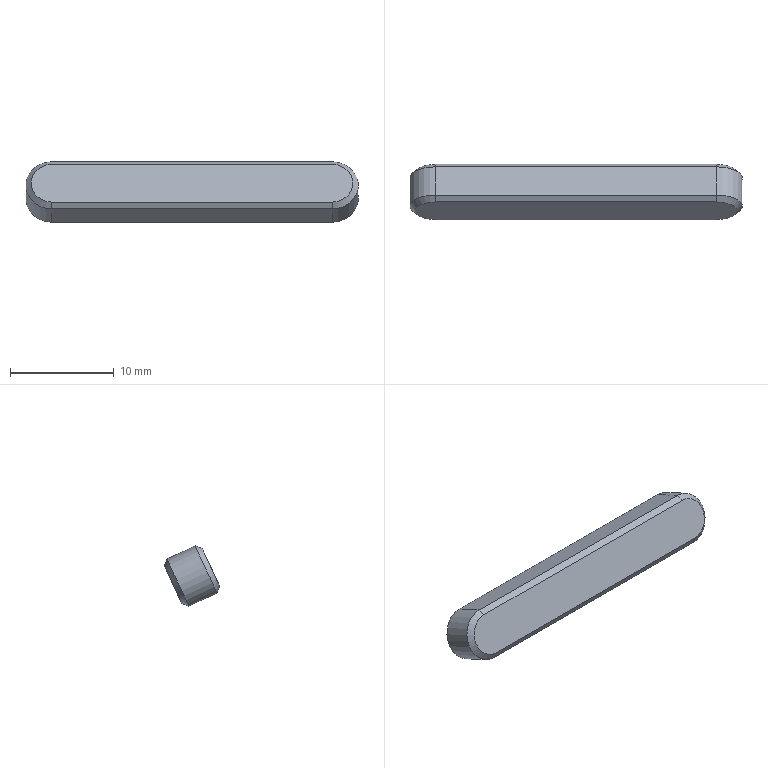Component | NX | KEY | 1 solid | 14 faces | box 32 x 5.32 x 5.8 mm | volume 601 mm3 | plane 8 | cone 4 | cylinder 2 | commonest cylinder face diameters 5 x2
STEP:
#1=CARTESIAN_POINT('',(0.,0.,0.));
#2=DIRECTION('',(0.,0.,1.));
#3=DIRECTION('',(1.,0.,0.));
#4=AXIS2_PLACEMENT_3D('',#1,#2,#3);
#5=CARTESIAN_POINT('',(56.5,-40.54,76.297));
#6=VERTEX_POINT('',#5);
#7=CARTESIAN_POINT('',(56.5,-43.259,77.565));
#8=VERTEX_POINT('',#7);
#9=CARTESIAN_POINT('',(56.5,-40.087,76.085));
#10=DIRECTION('',(0.,-0.9063,0.4226));
#11=VECTOR('',#10,1.);
#12=LINE('',#9,#11);
#13=CARTESIAN_POINT('',(56.5,-39.031,78.351));
#14=DIRECTION('',(0.,-0.9063,0.4226));
#15=DIRECTION('',(-1.,0.,0.));
#16=AXIS2_PLACEMENT_3D('',#13,#14,#15);
#17=CYLINDRICAL_SURFACE('',#16,2.5);
#18=CARTESIAN_POINT('',(1.571,-0.));
#19=DIRECTION('',(0.,1.));
#20=VECTOR('',#19,1.);
#21=LINE('',#18,#20);
#22=(GEOMETRIC_REPRESENTATION_CONTEXT(2)PARAMETRIC_REPRESENTATION_CONTEXT()REPRESENTATION_CONTEXT('',''));
#23=DEFINITIONAL_REPRESENTATION('',(#21),#22);
#24=PCURVE('',#17,#23);
#25=CARTESIAN_POINT('',(83.5,-40.087,76.085));
#26=DIRECTION('',(-0.,0.4226,0.9063));
#27=DIRECTION('',(1.,0.,0.));
#28=AXIS2_PLACEMENT_3D('',#25,#26,#27);
#29=PLANE('',#28);
#30=CARTESIAN_POINT('',(-27.,0.));
#31=DIRECTION('',(-0.,-1.));
#32=VECTOR('',#31,1.);
#33=LINE('',#30,#32);
#34=(GEOMETRIC_REPRESENTATION_CONTEXT(2)PARAMETRIC_REPRESENTATION_CONTEXT()REPRESENTATION_CONTEXT('',''));
#35=DEFINITIONAL_REPRESENTATION('',(#33),#34);
#36=PCURVE('',#29,#35);
#37=SURFACE_CURVE('',#12,(#24,#36),.PCURVE_S1.);
#38=EDGE_CURVE('',#6,#8,#37,.T.);
#39=ORIENTED_EDGE('',*,*,#38,.T.);
#40=CARTESIAN_POINT('',(56.5,-41.146,82.096));
#41=VERTEX_POINT('',#40);
#42=CARTESIAN_POINT('',(56.5,-42.203,79.83));
#43=DIRECTION('',(0.,0.9063,-0.4226));
#44=DIRECTION('',(1.,0.,0.));
#45=AXIS2_PLACEMENT_3D('',#42,#43,#44);
#46=CIRCLE('',#45,2.5);
#47=CARTESIAN_POINT('',(3.142,3.5));
#48=DIRECTION('',(-1.,0.));
#49=VECTOR('',#48,1.);
#50=LINE('',#47,#49);
#51=(GEOMETRIC_REPRESENTATION_CONTEXT(2)PARAMETRIC_REPRESENTATION_CONTEXT()REPRESENTATION_CONTEXT('',''));
#52=DEFINITIONAL_REPRESENTATION('',(#50),#51);
#53=PCURVE('',#17,#52);
#54=CARTESIAN_POINT('',(56.5,-42.203,79.83));
#55=DIRECTION('',(0.,0.9063,-0.4226));
#56=DIRECTION('',(1.,0.,0.));
#57=AXIS2_PLACEMENT_3D('',#54,#55,#56);
#58=CONICAL_SURFACE('',#57,2.5,0.7854);
#59=CARTESIAN_POINT('',(0.,0.));
#60=DIRECTION('',(1.,-0.));
#61=VECTOR('',#60,1.);
#62=LINE('',#59,#61);
#63=(GEOMETRIC_REPRESENTATION_CONTEXT(2)PARAMETRIC_REPRESENTATION_CONTEXT()REPRESENTATION_CONTEXT('',''));
#64=DEFINITIONAL_REPRESENTATION('',(#62),#63);
#65=PCURVE('',#58,#64);
#66=SURFACE_CURVE('',#46,(#53,#65),.PCURVE_S1.);
#67=EDGE_CURVE('',#8,#41,#66,.T.);
#68=ORIENTED_EDGE('',*,*,#67,.T.);
#69=CARTESIAN_POINT('',(56.5,-38.427,80.828));
#70=VERTEX_POINT('',#69);
#71=CARTESIAN_POINT('',(56.5,-37.974,80.617));
#72=DIRECTION('',(0.,-0.9063,0.4226));
#73=VECTOR('',#72,1.);
#74=LINE('',#71,#73);
#75=CARTESIAN_POINT('',(-1.571,-0.));
#76=DIRECTION('',(0.,1.));
#77=VECTOR('',#76,1.);
#78=LINE('',#75,#77);
#79=(GEOMETRIC_REPRESENTATION_CONTEXT(2)PARAMETRIC_REPRESENTATION_CONTEXT()REPRESENTATION_CONTEXT('',''));
#80=DEFINITIONAL_REPRESENTATION('',(#78),#79);
#81=PCURVE('',#17,#80);
#82=CARTESIAN_POINT('',(56.5,-37.974,80.617));
#83=DIRECTION('',(0.,-0.4226,-0.9063));
#84=DIRECTION('',(0.,0.9063,-0.4226));
#85=AXIS2_PLACEMENT_3D('',#82,#83,#84);
#86=PLANE('',#85);
#87=CARTESIAN_POINT('',(0.,0.));
#88=DIRECTION('',(-1.,0.));
#89=VECTOR('',#88,1.);
#90=LINE('',#87,#89);
#91=(GEOMETRIC_REPRESENTATION_CONTEXT(2)PARAMETRIC_REPRESENTATION_CONTEXT()REPRESENTATION_CONTEXT('',''));
#92=DEFINITIONAL_REPRESENTATION('',(#90),#91);
#93=PCURVE('',#86,#92);
#94=SURFACE_CURVE('',#74,(#81,#93),.PCURVE_S1.);
#95=EDGE_CURVE('',#70,#41,#94,.T.);
#96=ORIENTED_EDGE('',*,*,#95,.F.);
#97=CARTESIAN_POINT('',(56.5,-39.484,78.563));
#98=DIRECTION('',(0.,-0.9063,0.4226));
#99=DIRECTION('',(1.,0.,0.));
#100=AXIS2_PLACEMENT_3D('',#97,#98,#99);
#101=CIRCLE('',#100,2.5);
#102=CARTESIAN_POINT('',(-3.142,0.5));
#103=DIRECTION('',(1.,0.));
#104=VECTOR('',#103,1.);
#105=LINE('',#102,#104);
#106=(GEOMETRIC_REPRESENTATION_CONTEXT(2)PARAMETRIC_REPRESENTATION_CONTEXT()REPRESENTATION_CONTEXT('',''));
#107=DEFINITIONAL_REPRESENTATION('',(#105),#106);
#108=PCURVE('',#17,#107);
#109=CARTESIAN_POINT('',(56.5,-39.031,78.351));
#110=DIRECTION('',(0.,-0.9063,0.4226));
#111=DIRECTION('',(-1.,0.,0.));
#112=AXIS2_PLACEMENT_3D('',#109,#110,#111);
#113=CONICAL_SURFACE('',#112,2.,0.7854);
#114=CARTESIAN_POINT('',(-3.142,0.5));
#115=DIRECTION('',(1.,0.));
#116=VECTOR('',#115,1.);
#117=LINE('',#114,#116);
#118=(GEOMETRIC_REPRESENTATION_CONTEXT(2)PARAMETRIC_REPRESENTATION_CONTEXT()REPRESENTATION_CONTEXT('',''));
#119=DEFINITIONAL_REPRESENTATION('',(#117),#118);
#120=PCURVE('',#113,#119);
#121=SURFACE_CURVE('',#101,(#108,#120),.PCURVE_S1.);
#122=EDGE_CURVE('',#70,#6,#121,.T.);
#123=ORIENTED_EDGE('',*,*,#122,.T.);
#124=EDGE_LOOP('',(#39,#68,#96,#123));
#125=FACE_BOUND('',#124,.T.);
#126=ADVANCED_FACE('',(#125),#17,.T.);
#127=ORIENTED_EDGE('',*,*,#95,.T.);
#128=CARTESIAN_POINT('',(83.5,-41.146,82.096));
#129=VERTEX_POINT('',#128);
#130=CARTESIAN_POINT('',(56.5,-41.146,82.096));
#131=DIRECTION('',(1.,0.,0.));
#132=VECTOR('',#131,1.);
#133=LINE('',#130,#132);
#134=CARTESIAN_POINT('',(-3.5,0.));
#135=DIRECTION('',(0.,1.));
#136=VECTOR('',#135,1.);
#137=LINE('',#134,#136);
#138=(GEOMETRIC_REPRESENTATION_CONTEXT(2)PARAMETRIC_REPRESENTATION_CONTEXT()REPRESENTATION_CONTEXT('',''));
#139=DEFINITIONAL_REPRESENTATION('',(#137),#138);
#140=PCURVE('',#86,#139);
#141=CARTESIAN_POINT('',(56.5,-41.146,82.096));
#142=DIRECTION('',(0.,0.342,-0.9397));
#143=DIRECTION('',(1.,0.,0.));
#144=AXIS2_PLACEMENT_3D('',#141,#142,#143);
#145=PLANE('',#144);
#146=CARTESIAN_POINT('',(0.,0.));
#147=DIRECTION('',(1.,0.));
#148=VECTOR('',#147,1.);
#149=LINE('',#146,#148);
#150=(GEOMETRIC_REPRESENTATION_CONTEXT(2)PARAMETRIC_REPRESENTATION_CONTEXT()REPRESENTATION_CONTEXT('',''));
#151=DEFINITIONAL_REPRESENTATION('',(#149),#150);
#152=PCURVE('',#145,#151);
#153=SURFACE_CURVE('',#133,(#140,#152),.PCURVE_S1.);
#154=EDGE_CURVE('',#41,#129,#153,.T.);
#155=ORIENTED_EDGE('',*,*,#154,.T.);
#156=CARTESIAN_POINT('',(83.5,-38.427,80.828));
#157=VERTEX_POINT('',#156);
#158=CARTESIAN_POINT('',(83.5,-37.974,80.617));
#159=DIRECTION('',(0.,-0.9063,0.4226));
#160=VECTOR('',#159,1.);
#161=LINE('',#158,#160);
#162=CARTESIAN_POINT('',(0.,27.));
#163=DIRECTION('',(-1.,0.));
#164=VECTOR('',#163,1.);
#165=LINE('',#162,#164);
#166=(GEOMETRIC_REPRESENTATION_CONTEXT(2)PARAMETRIC_REPRESENTATION_CONTEXT()REPRESENTATION_CONTEXT('',''));
#167=DEFINITIONAL_REPRESENTATION('',(#165),#166);
#168=PCURVE('',#86,#167);
#169=CARTESIAN_POINT('',(83.5,-39.031,78.351));
#170=DIRECTION('',(0.,-0.9063,0.4226));
#171=DIRECTION('',(-1.,0.,0.));
#172=AXIS2_PLACEMENT_3D('',#169,#170,#171);
#173=CYLINDRICAL_SURFACE('',#172,2.5);
#174=CARTESIAN_POINT('',(4.712,-0.));
#175=DIRECTION('',(0.,1.));
#176=VECTOR('',#175,1.);
#177=LINE('',#174,#176);
#178=(GEOMETRIC_REPRESENTATION_CONTEXT(2)PARAMETRIC_REPRESENTATION_CONTEXT()REPRESENTATION_CONTEXT('',''));
#179=DEFINITIONAL_REPRESENTATION('',(#177),#178);
#180=PCURVE('',#173,#179);
#181=SURFACE_CURVE('',#161,(#168,#180),.PCURVE_S1.);
#182=EDGE_CURVE('',#157,#129,#181,.T.);
#183=ORIENTED_EDGE('',*,*,#182,.F.);
#184=CARTESIAN_POINT('',(56.5,-38.427,80.828));
#185=DIRECTION('',(-1.,0.,0.));
#186=VECTOR('',#185,1.);
#187=LINE('',#184,#186);
#188=CARTESIAN_POINT('',(-0.5,0.));
#189=DIRECTION('',(0.,-1.));
#190=VECTOR('',#189,1.);
#191=LINE('',#188,#190);
#192=(GEOMETRIC_REPRESENTATION_CONTEXT(2)PARAMETRIC_REPRESENTATION_CONTEXT()REPRESENTATION_CONTEXT('',''));
#193=DEFINITIONAL_REPRESENTATION('',(#191),#192);
#194=PCURVE('',#86,#193);
#195=CARTESIAN_POINT('',(56.5,-38.185,80.164));
#196=DIRECTION('',(0.,0.9397,0.342));
#197=DIRECTION('',(-1.,0.,0.));
#198=AXIS2_PLACEMENT_3D('',#195,#196,#197);
#199=PLANE('',#198);
#200=CARTESIAN_POINT('',(0.,0.7071));
#201=DIRECTION('',(1.,0.));
#202=VECTOR('',#201,1.);
#203=LINE('',#200,#202);
#204=(GEOMETRIC_REPRESENTATION_CONTEXT(2)PARAMETRIC_REPRESENTATION_CONTEXT()REPRESENTATION_CONTEXT('',''));
#205=DEFINITIONAL_REPRESENTATION('',(#203),#204);
#206=PCURVE('',#199,#205);
#207=SURFACE_CURVE('',#187,(#194,#206),.PCURVE_S1.);
#208=EDGE_CURVE('',#157,#70,#207,.T.);
#209=ORIENTED_EDGE('',*,*,#208,.T.);
#210=EDGE_LOOP('',(#127,#155,#183,#209));
#211=FACE_BOUND('',#210,.T.);
#212=ADVANCED_FACE('',(#211),#86,.F.);
#213=ORIENTED_EDGE('',*,*,#182,.T.);
#214=CARTESIAN_POINT('',(83.5,-43.259,77.565));
#215=VERTEX_POINT('',#214);
#216=CARTESIAN_POINT('',(83.5,-42.203,79.83));
#217=DIRECTION('',(0.,0.9063,-0.4226));
#218=DIRECTION('',(1.,0.,0.));
#219=AXIS2_PLACEMENT_3D('',#216,#217,#218);
#220=CIRCLE('',#219,2.5);
#221=CARTESIAN_POINT('',(9.425,3.5));
#222=DIRECTION('',(-1.,0.));
#223=VECTOR('',#222,1.);
#224=LINE('',#221,#223);
#225=(GEOMETRIC_REPRESENTATION_CONTEXT(2)PARAMETRIC_REPRESENTATION_CONTEXT()REPRESENTATION_CONTEXT('',''));
#226=DEFINITIONAL_REPRESENTATION('',(#224),#225);
#227=PCURVE('',#173,#226);
#228=CARTESIAN_POINT('',(83.5,-42.203,79.83));
#229=DIRECTION('',(0.,0.9063,-0.4226));
#230=DIRECTION('',(1.,0.,0.));
#231=AXIS2_PLACEMENT_3D('',#228,#229,#230);
#232=CONICAL_SURFACE('',#231,2.5,0.7854);
#233=CARTESIAN_POINT('',(0.,-0.));
#234=DIRECTION('',(1.,0.));
#235=VECTOR('',#234,1.);
#236=LINE('',#233,#235);
#237=(GEOMETRIC_REPRESENTATION_CONTEXT(2)PARAMETRIC_REPRESENTATION_CONTEXT()REPRESENTATION_CONTEXT('',''));
#238=DEFINITIONAL_REPRESENTATION('',(#236),#237);
#239=PCURVE('',#232,#238);
#240=SURFACE_CURVE('',#220,(#227,#239),.PCURVE_S1.);
#241=EDGE_CURVE('',#129,#215,#240,.T.);
#242=ORIENTED_EDGE('',*,*,#241,.T.);
#243=CARTESIAN_POINT('',(83.5,-40.54,76.297));
#244=VERTEX_POINT('',#243);
#245=CARTESIAN_POINT('',(83.5,-40.087,76.085));
#246=DIRECTION('',(0.,-0.9063,0.4226));
#247=VECTOR('',#246,1.);
#248=LINE('',#245,#247);
#249=CARTESIAN_POINT('',(1.571,-0.));
#250=DIRECTION('',(0.,1.));
#251=VECTOR('',#250,1.);
#252=LINE('',#249,#251);
#253=(GEOMETRIC_REPRESENTATION_CONTEXT(2)PARAMETRIC_REPRESENTATION_CONTEXT()REPRESENTATION_CONTEXT('',''));
#254=DEFINITIONAL_REPRESENTATION('',(#252),#253);
#255=PCURVE('',#173,#254);
#256=CARTESIAN_POINT('',(0.,0.));
#257=DIRECTION('',(-0.,-1.));
#258=VECTOR('',#257,1.);
#259=LINE('',#256,#258);
#260=(GEOMETRIC_REPRESENTATION_CONTEXT(2)PARAMETRIC_REPRESENTATION_CONTEXT()REPRESENTATION_CONTEXT('',''));
#261=DEFINITIONAL_REPRESENTATION('',(#259),#260);
#262=PCURVE('',#29,#261);
#263=SURFACE_CURVE('',#248,(#255,#262),.PCURVE_S1.);
#264=EDGE_CURVE('',#244,#215,#263,.T.);
#265=ORIENTED_EDGE('',*,*,#264,.F.);
#266=CARTESIAN_POINT('',(83.5,-39.484,78.563));
#267=DIRECTION('',(0.,-0.9063,0.4226));
#268=DIRECTION('',(1.,0.,0.));
#269=AXIS2_PLACEMENT_3D('',#266,#267,#268);
#270=CIRCLE('',#269,2.5);
#271=CARTESIAN_POINT('',(-3.142,0.5));
#272=DIRECTION('',(1.,0.));
#273=VECTOR('',#272,1.);
#274=LINE('',#271,#273);
#275=(GEOMETRIC_REPRESENTATION_CONTEXT(2)PARAMETRIC_REPRESENTATION_CONTEXT()REPRESENTATION_CONTEXT('',''));
#276=DEFINITIONAL_REPRESENTATION('',(#274),#275);
#277=PCURVE('',#173,#276);
#278=CARTESIAN_POINT('',(83.5,-39.031,78.351));
#279=DIRECTION('',(0.,-0.9063,0.4226));
#280=DIRECTION('',(-1.,0.,0.));
#281=AXIS2_PLACEMENT_3D('',#278,#279,#280);
#282=CONICAL_SURFACE('',#281,2.,0.7854);
#283=CARTESIAN_POINT('',(-3.142,0.5));
#284=DIRECTION('',(1.,-0.));
#285=VECTOR('',#284,1.);
#286=LINE('',#283,#285);
#287=(GEOMETRIC_REPRESENTATION_CONTEXT(2)PARAMETRIC_REPRESENTATION_CONTEXT()REPRESENTATION_CONTEXT('',''));
#288=DEFINITIONAL_REPRESENTATION('',(#286),#287);
#289=PCURVE('',#282,#288);
#290=SURFACE_CURVE('',#270,(#277,#289),.PCURVE_S1.);
#291=EDGE_CURVE('',#244,#157,#290,.T.);
#292=ORIENTED_EDGE('',*,*,#291,.T.);
#293=EDGE_LOOP('',(#213,#242,#265,#292));
#294=FACE_BOUND('',#293,.T.);
#295=ADVANCED_FACE('',(#294),#173,.T.);
#296=ORIENTED_EDGE('',*,*,#264,.T.);
#297=CARTESIAN_POINT('',(83.5,-43.259,77.565));
#298=DIRECTION('',(-1.,-0.,-0.));
#299=VECTOR('',#298,1.);
#300=LINE('',#297,#299);
#301=CARTESIAN_POINT('',(-0.,-3.5));
#302=DIRECTION('',(-1.,0.));
#303=VECTOR('',#302,1.);
#304=LINE('',#301,#303);
#305=(GEOMETRIC_REPRESENTATION_CONTEXT(2)PARAMETRIC_REPRESENTATION_CONTEXT()REPRESENTATION_CONTEXT('',''));
#306=DEFINITIONAL_REPRESENTATION('',(#304),#305);
#307=PCURVE('',#29,#306);
#308=CARTESIAN_POINT('',(83.5,-43.259,77.565));
#309=DIRECTION('',(-0.,0.9397,0.342));
#310=DIRECTION('',(-1.,-0.,-0.));
#311=AXIS2_PLACEMENT_3D('',#308,#309,#310);
#312=PLANE('',#311);
#313=CARTESIAN_POINT('',(0.,0.));
#314=DIRECTION('',(1.,-0.));
#315=VECTOR('',#314,1.);
#316=LINE('',#313,#315);
#317=(GEOMETRIC_REPRESENTATION_CONTEXT(2)PARAMETRIC_REPRESENTATION_CONTEXT()REPRESENTATION_CONTEXT('',''));
#318=DEFINITIONAL_REPRESENTATION('',(#316),#317);
#319=PCURVE('',#312,#318);
#320=SURFACE_CURVE('',#300,(#307,#319),.PCURVE_S1.);
#321=EDGE_CURVE('',#215,#8,#320,.T.);
#322=ORIENTED_EDGE('',*,*,#321,.T.);
#323=ORIENTED_EDGE('',*,*,#38,.F.);
#324=CARTESIAN_POINT('',(83.5,-40.54,76.297));
#325=DIRECTION('',(1.,0.,0.));
#326=VECTOR('',#325,1.);
#327=LINE('',#324,#326);
#328=CARTESIAN_POINT('',(-0.,-0.5));
#329=DIRECTION('',(1.,-0.));
#330=VECTOR('',#329,1.);
#331=LINE('',#328,#330);
#332=(GEOMETRIC_REPRESENTATION_CONTEXT(2)PARAMETRIC_REPRESENTATION_CONTEXT()REPRESENTATION_CONTEXT('',''));
#333=DEFINITIONAL_REPRESENTATION('',(#331),#332);
#334=PCURVE('',#29,#333);
#335=CARTESIAN_POINT('',(56.5,-39.876,76.539));
#336=DIRECTION('',(0.,0.342,-0.9397));
#337=DIRECTION('',(1.,0.,0.));
#338=AXIS2_PLACEMENT_3D('',#335,#336,#337);
#339=PLANE('',#338);
#340=CARTESIAN_POINT('',(27.,0.7071));
#341=DIRECTION('',(1.,-0.));
#342=VECTOR('',#341,1.);
#343=LINE('',#340,#342);
#344=(GEOMETRIC_REPRESENTATION_CONTEXT(2)PARAMETRIC_REPRESENTATION_CONTEXT()REPRESENTATION_CONTEXT('',''));
#345=DEFINITIONAL_REPRESENTATION('',(#343),#344);
#346=PCURVE('',#339,#345);
#347=SURFACE_CURVE('',#327,(#334,#346),.PCURVE_S1.);
#348=EDGE_CURVE('',#6,#244,#347,.T.);
#349=ORIENTED_EDGE('',*,*,#348,.T.);
#350=EDGE_LOOP('',(#296,#322,#323,#349));
#351=FACE_BOUND('',#350,.T.);
#352=ADVANCED_FACE('',(#351),#29,.F.);
#353=CARTESIAN_POINT('',(83.5,-39.876,76.539));
#354=VERTEX_POINT('',#353);
#355=CARTESIAN_POINT('',(56.5,-39.876,76.539));
#356=VERTEX_POINT('',#355);
#357=CARTESIAN_POINT('',(56.5,-39.876,76.539));
#358=DIRECTION('',(-1.,-0.,-0.));
#359=VECTOR('',#358,1.);
#360=LINE('',#357,#359);
#361=CARTESIAN_POINT('',(56.5,-39.031,78.351));
#362=DIRECTION('',(0.,0.9063,-0.4226));
#363=DIRECTION('',(1.,0.,0.));
#364=AXIS2_PLACEMENT_3D('',#361,#362,#363);
#365=PLANE('',#364);
#366=CARTESIAN_POINT('',(0.,2.));
#367=DIRECTION('',(-1.,0.));
#368=VECTOR('',#367,1.);
#369=LINE('',#366,#368);
#370=(GEOMETRIC_REPRESENTATION_CONTEXT(2)PARAMETRIC_REPRESENTATION_CONTEXT()REPRESENTATION_CONTEXT('',''));
#371=DEFINITIONAL_REPRESENTATION('',(#369),#370);
#372=PCURVE('',#365,#371);
#373=CARTESIAN_POINT('',(0.,0.));
#374=DIRECTION('',(-1.,0.));
#375=VECTOR('',#374,1.);
#376=LINE('',#373,#375);
#377=(GEOMETRIC_REPRESENTATION_CONTEXT(2)PARAMETRIC_REPRESENTATION_CONTEXT()REPRESENTATION_CONTEXT('',''));
#378=DEFINITIONAL_REPRESENTATION('',(#376),#377);
#379=PCURVE('',#339,#378);
#380=SURFACE_CURVE('',#360,(#372,#379),.PCURVE_S1.);
#381=EDGE_CURVE('',#354,#356,#380,.T.);
#382=ORIENTED_EDGE('',*,*,#381,.T.);
#383=CARTESIAN_POINT('',(56.5,-38.185,80.164));
#384=VERTEX_POINT('',#383);
#385=CARTESIAN_POINT('',(56.5,-39.031,78.351));
#386=DIRECTION('',(0.,0.9063,-0.4226));
#387=DIRECTION('',(1.,0.,0.));
#388=AXIS2_PLACEMENT_3D('',#385,#386,#387);
#389=CIRCLE('',#388,2.);
#390=CARTESIAN_POINT('',(0.,0.));
#391=DIRECTION('',(1.,0.));
#392=AXIS2_PLACEMENT_2D('',#390,#391);
#393=CIRCLE('',#392,2.);
#394=(GEOMETRIC_REPRESENTATION_CONTEXT(2)PARAMETRIC_REPRESENTATION_CONTEXT()REPRESENTATION_CONTEXT('',''));
#395=DEFINITIONAL_REPRESENTATION('',(#393),#394);
#396=PCURVE('',#365,#395);
#397=CARTESIAN_POINT('',(3.142,-0.));
#398=DIRECTION('',(-1.,0.));
#399=VECTOR('',#398,1.);
#400=LINE('',#397,#399);
#401=(GEOMETRIC_REPRESENTATION_CONTEXT(2)PARAMETRIC_REPRESENTATION_CONTEXT()REPRESENTATION_CONTEXT('',''));
#402=DEFINITIONAL_REPRESENTATION('',(#400),#401);
#403=PCURVE('',#113,#402);
#404=SURFACE_CURVE('',#389,(#396,#403),.PCURVE_S1.);
#405=EDGE_CURVE('',#356,#384,#404,.T.);
#406=ORIENTED_EDGE('',*,*,#405,.T.);
#407=CARTESIAN_POINT('',(83.5,-38.185,80.164));
#408=VERTEX_POINT('',#407);
#409=CARTESIAN_POINT('',(83.5,-38.185,80.164));
#410=DIRECTION('',(1.,0.,0.));
#411=VECTOR('',#410,1.);
#412=LINE('',#409,#411);
#413=CARTESIAN_POINT('',(27.,-2.));
#414=DIRECTION('',(1.,0.));
#415=VECTOR('',#414,1.);
#416=LINE('',#413,#415);
#417=(GEOMETRIC_REPRESENTATION_CONTEXT(2)PARAMETRIC_REPRESENTATION_CONTEXT()REPRESENTATION_CONTEXT('',''));
#418=DEFINITIONAL_REPRESENTATION('',(#416),#417);
#419=PCURVE('',#365,#418);
#420=CARTESIAN_POINT('',(-27.,0.));
#421=DIRECTION('',(-1.,0.));
#422=VECTOR('',#421,1.);
#423=LINE('',#420,#422);
#424=(GEOMETRIC_REPRESENTATION_CONTEXT(2)PARAMETRIC_REPRESENTATION_CONTEXT()REPRESENTATION_CONTEXT('',''));
#425=DEFINITIONAL_REPRESENTATION('',(#423),#424);
#426=PCURVE('',#199,#425);
#427=SURFACE_CURVE('',#412,(#419,#426),.PCURVE_S1.);
#428=EDGE_CURVE('',#384,#408,#427,.T.);
#429=ORIENTED_EDGE('',*,*,#428,.T.);
#430=CARTESIAN_POINT('',(83.5,-39.031,78.351));
#431=DIRECTION('',(0.,0.9063,-0.4226));
#432=DIRECTION('',(1.,0.,0.));
#433=AXIS2_PLACEMENT_3D('',#430,#431,#432);
#434=CIRCLE('',#433,2.);
#435=CARTESIAN_POINT('',(27.,0.));
#436=DIRECTION('',(1.,0.));
#437=AXIS2_PLACEMENT_2D('',#435,#436);
#438=CIRCLE('',#437,2.);
#439=(GEOMETRIC_REPRESENTATION_CONTEXT(2)PARAMETRIC_REPRESENTATION_CONTEXT()REPRESENTATION_CONTEXT('',''));
#440=DEFINITIONAL_REPRESENTATION('',(#438),#439);
#441=PCURVE('',#365,#440);
#442=CARTESIAN_POINT('',(9.425,-0.));
#443=DIRECTION('',(-1.,0.));
#444=VECTOR('',#443,1.);
#445=LINE('',#442,#444);
#446=(GEOMETRIC_REPRESENTATION_CONTEXT(2)PARAMETRIC_REPRESENTATION_CONTEXT()REPRESENTATION_CONTEXT('',''));
#447=DEFINITIONAL_REPRESENTATION('',(#445),#446);
#448=PCURVE('',#282,#447);
#449=SURFACE_CURVE('',#434,(#441,#448),.PCURVE_S1.);
#450=EDGE_CURVE('',#408,#354,#449,.T.);
#451=ORIENTED_EDGE('',*,*,#450,.T.);
#452=EDGE_LOOP('',(#382,#406,#429,#451));
#453=FACE_BOUND('',#452,.T.);
#454=ADVANCED_FACE('',(#453),#365,.T.);
#455=CARTESIAN_POINT('',(83.5,-41.811,81.854));
#456=VERTEX_POINT('',#455);
#457=CARTESIAN_POINT('',(56.5,-41.811,81.854));
#458=VERTEX_POINT('',#457);
#459=CARTESIAN_POINT('',(56.5,-41.811,81.854));
#460=DIRECTION('',(-1.,0.,0.));
#461=VECTOR('',#460,1.);
#462=LINE('',#459,#461);
#463=CARTESIAN_POINT('',(56.5,-42.656,80.042));
#464=DIRECTION('',(0.,0.9063,-0.4226));
#465=DIRECTION('',(1.,0.,0.));
#466=AXIS2_PLACEMENT_3D('',#463,#464,#465);
#467=PLANE('',#466);
#468=CARTESIAN_POINT('',(0.,-2.));
#469=DIRECTION('',(-1.,0.));
#470=VECTOR('',#469,1.);
#471=LINE('',#468,#470);
#472=(GEOMETRIC_REPRESENTATION_CONTEXT(2)PARAMETRIC_REPRESENTATION_CONTEXT()REPRESENTATION_CONTEXT('',''));
#473=DEFINITIONAL_REPRESENTATION('',(#471),#472);
#474=PCURVE('',#467,#473);
#475=CARTESIAN_POINT('',(0.,0.7071));
#476=DIRECTION('',(-1.,0.));
#477=VECTOR('',#476,1.);
#478=LINE('',#475,#477);
#479=(GEOMETRIC_REPRESENTATION_CONTEXT(2)PARAMETRIC_REPRESENTATION_CONTEXT()REPRESENTATION_CONTEXT('',''));
#480=DEFINITIONAL_REPRESENTATION('',(#478),#479);
#481=PCURVE('',#145,#480);
#482=SURFACE_CURVE('',#462,(#474,#481),.PCURVE_S1.);
#483=EDGE_CURVE('',#456,#458,#482,.T.);
#484=ORIENTED_EDGE('',*,*,#483,.T.);
#485=CARTESIAN_POINT('',(56.5,-43.501,78.229));
#486=VERTEX_POINT('',#485);
#487=CARTESIAN_POINT('',(56.5,-42.656,80.042));
#488=DIRECTION('',(0.,-0.9063,0.4226));
#489=DIRECTION('',(1.,0.,0.));
#490=AXIS2_PLACEMENT_3D('',#487,#488,#489);
#491=CIRCLE('',#490,2.);
#492=CARTESIAN_POINT('',(2.,0.));
#493=CARTESIAN_POINT('',(2.,-3.464));
#494=CARTESIAN_POINT('',(-1.,-1.732));
#495=CARTESIAN_POINT('',(-4.,-0.));
#496=CARTESIAN_POINT('',(-1.,1.732));
#497=CARTESIAN_POINT('',(2.,3.464));
#498=CARTESIAN_POINT('',(2.,0.));
#499=(BOUNDED_CURVE()B_SPLINE_CURVE(2,(#492,#493,#494,#495,#496,#497,#498),.UNSPECIFIED.,.T.,.F.)B_SPLINE_CURVE_WITH_KNOTS((1,2,2,2,2,1),(-2.094,0.,2.094,4.189,6.283,8.378),.UNSPECIFIED.)CURVE()GEOMETRIC_REPRESENTATION_ITEM()RATIONAL_B_SPLINE_CURVE((1.,0.5,1.,0.5,1.,0.5,1.))REPRESENTATION_ITEM(''));
#500=(GEOMETRIC_REPRESENTATION_CONTEXT(2)PARAMETRIC_REPRESENTATION_CONTEXT()REPRESENTATION_CONTEXT('',''));
#501=DEFINITIONAL_REPRESENTATION('',(#499),#500);
#502=PCURVE('',#467,#501);
#503=CARTESIAN_POINT('',(6.283,-0.5));
#504=DIRECTION('',(-1.,0.));
#505=VECTOR('',#504,1.);
#506=LINE('',#503,#505);
#507=(GEOMETRIC_REPRESENTATION_CONTEXT(2)PARAMETRIC_REPRESENTATION_CONTEXT()REPRESENTATION_CONTEXT('',''));
#508=DEFINITIONAL_REPRESENTATION('',(#506),#507);
#509=PCURVE('',#58,#508);
#510=SURFACE_CURVE('',#491,(#502,#509),.PCURVE_S1.);
#511=EDGE_CURVE('',#458,#486,#510,.T.);
#512=ORIENTED_EDGE('',*,*,#511,.T.);
#513=CARTESIAN_POINT('',(83.5,-43.501,78.229));
#514=VERTEX_POINT('',#513);
#515=CARTESIAN_POINT('',(56.5,-43.501,78.229));
#516=DIRECTION('',(1.,0.,0.));
#517=VECTOR('',#516,1.);
#518=LINE('',#515,#517);
#519=CARTESIAN_POINT('',(0.,2.));
#520=DIRECTION('',(1.,-0.));
#521=VECTOR('',#520,1.);
#522=LINE('',#519,#521);
#523=(GEOMETRIC_REPRESENTATION_CONTEXT(2)PARAMETRIC_REPRESENTATION_CONTEXT()REPRESENTATION_CONTEXT('',''));
#524=DEFINITIONAL_REPRESENTATION('',(#522),#523);
#525=PCURVE('',#467,#524);
#526=CARTESIAN_POINT('',(27.,0.7071));
#527=DIRECTION('',(-1.,0.));
#528=VECTOR('',#527,1.);
#529=LINE('',#526,#528);
#530=(GEOMETRIC_REPRESENTATION_CONTEXT(2)PARAMETRIC_REPRESENTATION_CONTEXT()REPRESENTATION_CONTEXT('',''));
#531=DEFINITIONAL_REPRESENTATION('',(#529),#530);
#532=PCURVE('',#312,#531);
#533=SURFACE_CURVE('',#518,(#525,#532),.PCURVE_S1.);
#534=EDGE_CURVE('',#486,#514,#533,.T.);
#535=ORIENTED_EDGE('',*,*,#534,.T.);
#536=CARTESIAN_POINT('',(83.5,-42.656,80.042));
#537=DIRECTION('',(0.,-0.9063,0.4226));
#538=DIRECTION('',(1.,0.,0.));
#539=AXIS2_PLACEMENT_3D('',#536,#537,#538);
#540=CIRCLE('',#539,2.);
#541=CARTESIAN_POINT('',(29.,0.));
#542=CARTESIAN_POINT('',(29.,-3.464));
#543=CARTESIAN_POINT('',(26.,-1.732));
#544=CARTESIAN_POINT('',(23.,-0.));
#545=CARTESIAN_POINT('',(26.,1.732));
#546=CARTESIAN_POINT('',(29.,3.464));
#547=CARTESIAN_POINT('',(29.,0.));
#548=(BOUNDED_CURVE()B_SPLINE_CURVE(2,(#541,#542,#543,#544,#545,#546,#547),.UNSPECIFIED.,.T.,.F.)B_SPLINE_CURVE_WITH_KNOTS((1,2,2,2,2,1),(-2.094,0.,2.094,4.189,6.283,8.378),.UNSPECIFIED.)CURVE()GEOMETRIC_REPRESENTATION_ITEM()RATIONAL_B_SPLINE_CURVE((1.,0.5,1.,0.5,1.,0.5,1.))REPRESENTATION_ITEM(''));
#549=(GEOMETRIC_REPRESENTATION_CONTEXT(2)PARAMETRIC_REPRESENTATION_CONTEXT()REPRESENTATION_CONTEXT('',''));
#550=DEFINITIONAL_REPRESENTATION('',(#548),#549);
#551=PCURVE('',#467,#550);
#552=CARTESIAN_POINT('',(12.566,-0.5));
#553=DIRECTION('',(-1.,-0.));
#554=VECTOR('',#553,1.);
#555=LINE('',#552,#554);
#556=(GEOMETRIC_REPRESENTATION_CONTEXT(2)PARAMETRIC_REPRESENTATION_CONTEXT()REPRESENTATION_CONTEXT('',''));
#557=DEFINITIONAL_REPRESENTATION('',(#555),#556);
#558=PCURVE('',#232,#557);
#559=SURFACE_CURVE('',#540,(#551,#558),.PCURVE_S1.);
#560=EDGE_CURVE('',#514,#456,#559,.T.);
#561=ORIENTED_EDGE('',*,*,#560,.T.);
#562=EDGE_LOOP('',(#484,#512,#535,#561));
#563=FACE_BOUND('',#562,.T.);
#564=ADVANCED_FACE('',(#563),#467,.F.);
#565=CARTESIAN_POINT('',(83.5,-41.811,81.854));
#566=DIRECTION('',(0.,0.9397,0.342));
#567=VECTOR('',#566,1.);
#568=LINE('',#565,#567);
#569=CARTESIAN_POINT('',(4.712,-0.5));
#570=DIRECTION('',(0.,1.));
#571=VECTOR('',#570,1.);
#572=LINE('',#569,#571);
#573=(GEOMETRIC_REPRESENTATION_CONTEXT(2)PARAMETRIC_REPRESENTATION_CONTEXT()REPRESENTATION_CONTEXT('',''));
#574=DEFINITIONAL_REPRESENTATION('',(#572),#573);
#575=PCURVE('',#232,#574);
#576=CARTESIAN_POINT('',(27.,0.7071));
#577=DIRECTION('',(0.,-1.));
#578=VECTOR('',#577,1.);
#579=LINE('',#576,#578);
#580=(GEOMETRIC_REPRESENTATION_CONTEXT(2)PARAMETRIC_REPRESENTATION_CONTEXT()REPRESENTATION_CONTEXT('',''));
#581=DEFINITIONAL_REPRESENTATION('',(#579),#580);
#582=PCURVE('',#145,#581);
#583=SURFACE_CURVE('',#568,(#575,#582),.PCURVE_S1.);
#584=EDGE_CURVE('',#456,#129,#583,.T.);
#585=ORIENTED_EDGE('',*,*,#584,.F.);
#586=ORIENTED_EDGE('',*,*,#560,.F.);
#587=CARTESIAN_POINT('',(83.5,-43.259,77.565));
#588=DIRECTION('',(0.,-0.342,0.9397));
#589=VECTOR('',#588,1.);
#590=LINE('',#587,#589);
#591=CARTESIAN_POINT('',(7.854,-0.));
#592=DIRECTION('',(0.,-1.));
#593=VECTOR('',#592,1.);
#594=LINE('',#591,#593);
#595=(GEOMETRIC_REPRESENTATION_CONTEXT(2)PARAMETRIC_REPRESENTATION_CONTEXT()REPRESENTATION_CONTEXT('',''));
#596=DEFINITIONAL_REPRESENTATION('',(#594),#595);
#597=PCURVE('',#232,#596);
#598=CARTESIAN_POINT('',(0.,0.));
#599=DIRECTION('',(-0.,1.));
#600=VECTOR('',#599,1.);
#601=LINE('',#598,#600);
#602=(GEOMETRIC_REPRESENTATION_CONTEXT(2)PARAMETRIC_REPRESENTATION_CONTEXT()REPRESENTATION_CONTEXT('',''));
#603=DEFINITIONAL_REPRESENTATION('',(#601),#602);
#604=PCURVE('',#312,#603);
#605=SURFACE_CURVE('',#590,(#597,#604),.PCURVE_S1.);
#606=EDGE_CURVE('',#215,#514,#605,.T.);
#607=ORIENTED_EDGE('',*,*,#606,.F.);
#608=ORIENTED_EDGE('',*,*,#241,.F.);
#609=EDGE_LOOP('',(#585,#586,#607,#608));
#610=FACE_BOUND('',#609,.T.);
#611=ADVANCED_FACE('',(#610),#232,.T.);
#612=ORIENTED_EDGE('',*,*,#606,.T.);
#613=ORIENTED_EDGE('',*,*,#534,.F.);
#614=CARTESIAN_POINT('',(56.5,-43.259,77.565));
#615=DIRECTION('',(0.,-0.342,0.9397));
#616=VECTOR('',#615,1.);
#617=LINE('',#614,#616);
#618=CARTESIAN_POINT('',(27.,0.));
#619=DIRECTION('',(-0.,1.));
#620=VECTOR('',#619,1.);
#621=LINE('',#618,#620);
#622=(GEOMETRIC_REPRESENTATION_CONTEXT(2)PARAMETRIC_REPRESENTATION_CONTEXT()REPRESENTATION_CONTEXT('',''));
#623=DEFINITIONAL_REPRESENTATION('',(#621),#622);
#624=PCURVE('',#312,#623);
#625=CARTESIAN_POINT('',(1.571,-0.));
#626=DIRECTION('',(0.,-1.));
#627=VECTOR('',#626,1.);
#628=LINE('',#625,#627);
#629=(GEOMETRIC_REPRESENTATION_CONTEXT(2)PARAMETRIC_REPRESENTATION_CONTEXT()REPRESENTATION_CONTEXT('',''));
#630=DEFINITIONAL_REPRESENTATION('',(#628),#629);
#631=PCURVE('',#58,#630);
#632=SURFACE_CURVE('',#617,(#624,#631),.PCURVE_S1.);
#633=EDGE_CURVE('',#8,#486,#632,.T.);
#634=ORIENTED_EDGE('',*,*,#633,.F.);
#635=ORIENTED_EDGE('',*,*,#321,.F.);
#636=EDGE_LOOP('',(#612,#613,#634,#635));
#637=FACE_BOUND('',#636,.T.);
#638=ADVANCED_FACE('',(#637),#312,.F.);
#639=ORIENTED_EDGE('',*,*,#584,.T.);
#640=ORIENTED_EDGE('',*,*,#154,.F.);
#641=CARTESIAN_POINT('',(56.5,-41.811,81.854));
#642=DIRECTION('',(0.,0.9397,0.342));
#643=VECTOR('',#642,1.);
#644=LINE('',#641,#643);
#645=CARTESIAN_POINT('',(0.,0.7071));
#646=DIRECTION('',(0.,-1.));
#647=VECTOR('',#646,1.);
#648=LINE('',#645,#647);
#649=(GEOMETRIC_REPRESENTATION_CONTEXT(2)PARAMETRIC_REPRESENTATION_CONTEXT()REPRESENTATION_CONTEXT('',''));
#650=DEFINITIONAL_REPRESENTATION('',(#648),#649);
#651=PCURVE('',#145,#650);
#652=CARTESIAN_POINT('',(4.712,-0.5));
#653=DIRECTION('',(0.,1.));
#654=VECTOR('',#653,1.);
#655=LINE('',#652,#654);
#656=(GEOMETRIC_REPRESENTATION_CONTEXT(2)PARAMETRIC_REPRESENTATION_CONTEXT()REPRESENTATION_CONTEXT('',''));
#657=DEFINITIONAL_REPRESENTATION('',(#655),#656);
#658=PCURVE('',#58,#657);
#659=SURFACE_CURVE('',#644,(#651,#658),.PCURVE_S1.);
#660=EDGE_CURVE('',#458,#41,#659,.T.);
#661=ORIENTED_EDGE('',*,*,#660,.F.);
#662=ORIENTED_EDGE('',*,*,#483,.F.);
#663=EDGE_LOOP('',(#639,#640,#661,#662));
#664=FACE_BOUND('',#663,.T.);
#665=ADVANCED_FACE('',(#664),#145,.F.);
#666=ORIENTED_EDGE('',*,*,#633,.T.);
#667=ORIENTED_EDGE('',*,*,#511,.F.);
#668=ORIENTED_EDGE('',*,*,#660,.T.);
#669=ORIENTED_EDGE('',*,*,#67,.F.);
#670=EDGE_LOOP('',(#666,#667,#668,#669));
#671=FACE_BOUND('',#670,.T.);
#672=ADVANCED_FACE('',(#671),#58,.T.);
#673=CARTESIAN_POINT('',(83.5,-38.427,80.828));
#674=DIRECTION('',(0.,0.342,-0.9397));
#675=VECTOR('',#674,1.);
#676=LINE('',#673,#675);
#677=CARTESIAN_POINT('',(4.712,0.5));
#678=DIRECTION('',(0.,-1.));
#679=VECTOR('',#678,1.);
#680=LINE('',#677,#679);
#681=(GEOMETRIC_REPRESENTATION_CONTEXT(2)PARAMETRIC_REPRESENTATION_CONTEXT()REPRESENTATION_CONTEXT('',''));
#682=DEFINITIONAL_REPRESENTATION('',(#680),#681);
#683=PCURVE('',#282,#682);
#684=CARTESIAN_POINT('',(-27.,0.7071));
#685=DIRECTION('',(0.,-1.));
#686=VECTOR('',#685,1.);
#687=LINE('',#684,#686);
#688=(GEOMETRIC_REPRESENTATION_CONTEXT(2)PARAMETRIC_REPRESENTATION_CONTEXT()REPRESENTATION_CONTEXT('',''));
#689=DEFINITIONAL_REPRESENTATION('',(#687),#688);
#690=PCURVE('',#199,#689);
#691=SURFACE_CURVE('',#676,(#683,#690),.PCURVE_S1.);
#692=EDGE_CURVE('',#157,#408,#691,.T.);
#693=ORIENTED_EDGE('',*,*,#692,.F.);
#694=ORIENTED_EDGE('',*,*,#291,.F.);
#695=CARTESIAN_POINT('',(83.5,-39.876,76.539));
#696=DIRECTION('',(0.,-0.9397,-0.342));
#697=VECTOR('',#696,1.);
#698=LINE('',#695,#697);
#699=CARTESIAN_POINT('',(1.571,-0.));
#700=DIRECTION('',(0.,1.));
#701=VECTOR('',#700,1.);
#702=LINE('',#699,#701);
#703=(GEOMETRIC_REPRESENTATION_CONTEXT(2)PARAMETRIC_REPRESENTATION_CONTEXT()REPRESENTATION_CONTEXT('',''));
#704=DEFINITIONAL_REPRESENTATION('',(#702),#703);
#705=PCURVE('',#282,#704);
#706=CARTESIAN_POINT('',(27.,0.));
#707=DIRECTION('',(-0.,1.));
#708=VECTOR('',#707,1.);
#709=LINE('',#706,#708);
#710=(GEOMETRIC_REPRESENTATION_CONTEXT(2)PARAMETRIC_REPRESENTATION_CONTEXT()REPRESENTATION_CONTEXT('',''));
#711=DEFINITIONAL_REPRESENTATION('',(#709),#710);
#712=PCURVE('',#339,#711);
#713=SURFACE_CURVE('',#698,(#705,#712),.PCURVE_S1.);
#714=EDGE_CURVE('',#354,#244,#713,.T.);
#715=ORIENTED_EDGE('',*,*,#714,.F.);
#716=ORIENTED_EDGE('',*,*,#450,.F.);
#717=EDGE_LOOP('',(#693,#694,#715,#716));
#718=FACE_BOUND('',#717,.T.);
#719=ADVANCED_FACE('',(#718),#282,.T.);
#720=ORIENTED_EDGE('',*,*,#714,.T.);
#721=ORIENTED_EDGE('',*,*,#348,.F.);
#722=CARTESIAN_POINT('',(56.5,-39.876,76.539));
#723=DIRECTION('',(0.,-0.9397,-0.342));
#724=VECTOR('',#723,1.);
#725=LINE('',#722,#724);
#726=CARTESIAN_POINT('',(0.,0.));
#727=DIRECTION('',(-0.,1.));
#728=VECTOR('',#727,1.);
#729=LINE('',#726,#728);
#730=(GEOMETRIC_REPRESENTATION_CONTEXT(2)PARAMETRIC_REPRESENTATION_CONTEXT()REPRESENTATION_CONTEXT('',''));
#731=DEFINITIONAL_REPRESENTATION('',(#729),#730);
#732=PCURVE('',#339,#731);
#733=CARTESIAN_POINT('',(1.571,-0.));
#734=DIRECTION('',(0.,1.));
#735=VECTOR('',#734,1.);
#736=LINE('',#733,#735);
#737=(GEOMETRIC_REPRESENTATION_CONTEXT(2)PARAMETRIC_REPRESENTATION_CONTEXT()REPRESENTATION_CONTEXT('',''));
#738=DEFINITIONAL_REPRESENTATION('',(#736),#737);
#739=PCURVE('',#113,#738);
#740=SURFACE_CURVE('',#725,(#732,#739),.PCURVE_S1.);
#741=EDGE_CURVE('',#356,#6,#740,.T.);
#742=ORIENTED_EDGE('',*,*,#741,.F.);
#743=ORIENTED_EDGE('',*,*,#381,.F.);
#744=EDGE_LOOP('',(#720,#721,#742,#743));
#745=FACE_BOUND('',#744,.T.);
#746=ADVANCED_FACE('',(#745),#339,.T.);
#747=ORIENTED_EDGE('',*,*,#692,.T.);
#748=ORIENTED_EDGE('',*,*,#428,.F.);
#749=CARTESIAN_POINT('',(56.5,-38.427,80.828));
#750=DIRECTION('',(0.,0.342,-0.9397));
#751=VECTOR('',#750,1.);
#752=LINE('',#749,#751);
#753=CARTESIAN_POINT('',(0.,0.7071));
#754=DIRECTION('',(0.,-1.));
#755=VECTOR('',#754,1.);
#756=LINE('',#753,#755);
#757=(GEOMETRIC_REPRESENTATION_CONTEXT(2)PARAMETRIC_REPRESENTATION_CONTEXT()REPRESENTATION_CONTEXT('',''));
#758=DEFINITIONAL_REPRESENTATION('',(#756),#757);
#759=PCURVE('',#199,#758);
#760=CARTESIAN_POINT('',(-1.571,0.5));
#761=DIRECTION('',(0.,-1.));
#762=VECTOR('',#761,1.);
#763=LINE('',#760,#762);
#764=(GEOMETRIC_REPRESENTATION_CONTEXT(2)PARAMETRIC_REPRESENTATION_CONTEXT()REPRESENTATION_CONTEXT('',''));
#765=DEFINITIONAL_REPRESENTATION('',(#763),#764);
#766=PCURVE('',#113,#765);
#767=SURFACE_CURVE('',#752,(#759,#766),.PCURVE_S1.);
#768=EDGE_CURVE('',#70,#384,#767,.T.);
#769=ORIENTED_EDGE('',*,*,#768,.F.);
#770=ORIENTED_EDGE('',*,*,#208,.F.);
#771=EDGE_LOOP('',(#747,#748,#769,#770));
#772=FACE_BOUND('',#771,.T.);
#773=ADVANCED_FACE('',(#772),#199,.T.);
#774=ORIENTED_EDGE('',*,*,#741,.T.);
#775=ORIENTED_EDGE('',*,*,#122,.F.);
#776=ORIENTED_EDGE('',*,*,#768,.T.);
#777=ORIENTED_EDGE('',*,*,#405,.F.);
#778=EDGE_LOOP('',(#774,#775,#776,#777));
#779=FACE_BOUND('',#778,.T.);
#780=ADVANCED_FACE('',(#779),#113,.T.);
#781=CLOSED_SHELL('',(#126,#212,#295,#352,#454,#564,#611,#638,#665,#672,#719,#746,#773,#780));
#782=MANIFOLD_SOLID_BREP('',#781);
#783=(LENGTH_UNIT()NAMED_UNIT(*)SI_UNIT(.MILLI.,.METRE.));
#784=UNCERTAINTY_MEASURE_WITH_UNIT(LENGTH_MEASURE(0.0000001),#783,'','');
#785=(NAMED_UNIT(*)PLANE_ANGLE_UNIT()SI_UNIT($,.RADIAN.));
#786=(NAMED_UNIT(*)SI_UNIT($,.STERADIAN.)SOLID_ANGLE_UNIT());
#787=(GEOMETRIC_REPRESENTATION_CONTEXT(3)GLOBAL_UNCERTAINTY_ASSIGNED_CONTEXT((#784))GLOBAL_UNIT_ASSIGNED_CONTEXT((#783,#785,#786))REPRESENTATION_CONTEXT('',''));
#788=ADVANCED_BREP_SHAPE_REPRESENTATION('',(#4,#782),#787);